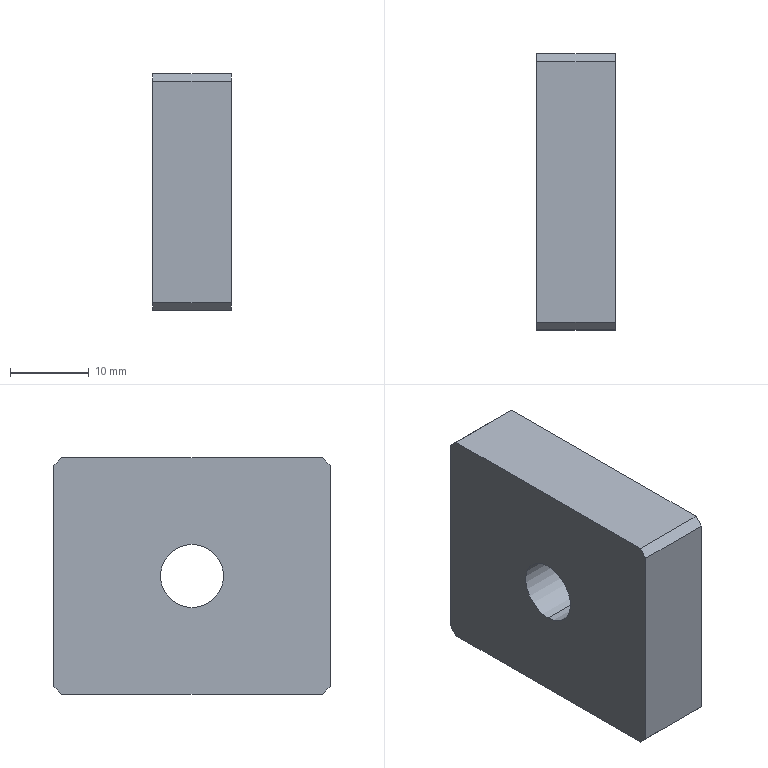Component | SolidWorks | XT-1-19-2-1 | 1 solid | 20 faces | box 10 x 35 x 30 mm | volume 9715 mm3 | plane 10 | cylinder 6 | cone 4 | commonest cylinder face diameters 3.3 x4 8 x2
build123d program:
from build123d import *

# Parameters (mm, degrees)
SKETCH1_W             = 30
SKETCH1_H             = 35
BOSS_EXTRUDE1_DEPTH   = 10
M4_TAPPED_HOLE1_D     = 3.3
M4_TAPPED_HOLE1_DEPTH = 15
M4_TAPPED_HOLE1_TIP   = 0.9914
M8_TAPPED_HOLE1_D     = 8
CHAMFER1_SIZE         = 1


with BuildPart() as part:
    # Sketch1 → Boss-Extrude1 (new body)
    with BuildSketch(Plane.XY):
        with Locations((15, -17.5)):
            Rectangle(SKETCH1_W, SKETCH1_H)
    extrude(amount=BOSS_EXTRUDE1_DEPTH)

    # M4 Tapped Hole1
    with Locations(Plane.ZY):
        with Locations((5, -7.5), (5, -27.5)):
            Hole(M4_TAPPED_HOLE1_D / 2, depth=M4_TAPPED_HOLE1_DEPTH)
            with Locations((0, 0, -(M4_TAPPED_HOLE1_DEPTH + M4_TAPPED_HOLE1_TIP / 2))):  # 118° drill point
                Cone(0, M4_TAPPED_HOLE1_D / 2, M4_TAPPED_HOLE1_TIP, mode=Mode.SUBTRACT)

    # M8 Tapped Hole1 (through all)
    with Locations(Plane.XY.offset(10)):
        with Locations((15, -17.5)):
            Hole(M8_TAPPED_HOLE1_D / 2)

    # Chamfer1
    chamfer1_edges = [part.edges().sort_by_distance(p)[0] for p in [
        (0, 0, 5),
        (30, 0, 5),
        (30, -35, 5),
        (0, -35, 5),
    ]]
    chamfer(chamfer1_edges, length=CHAMFER1_SIZE)


solid = part.part

# Placed as in the assembly
solid = solid.moved(Location((597.283, -101.115, -151), (0, -90, 0)))
STEP:
#1=COLOUR_RGB('',0.7922,0.8196,0.9333);
#2=FILL_AREA_STYLE_COLOUR('',#1);
#3=FILL_AREA_STYLE('',(#2));
#4=SURFACE_STYLE_FILL_AREA(#3);
#5=SURFACE_SIDE_STYLE('',(#4));
#6=SURFACE_STYLE_USAGE(.BOTH.,#5);
#7=PRESENTATION_STYLE_ASSIGNMENT((#6));
#8=CARTESIAN_POINT('',(23.515,-4.67,-5.512));
#9=VERTEX_POINT('',#8);
#10=CARTESIAN_POINT('',(23.515,-4.67,-5.197));
#11=VERTEX_POINT('',#10);
#12=CARTESIAN_POINT('',(23.515,-4.67,-5.354));
#13=DIRECTION('',(-1.,-0.,-0.));
#14=DIRECTION('',(0.,0.,1.));
#15=AXIS2_PLACEMENT_3D('',#12,#13,#14);
#16=CIRCLE('',#15,0.1575);
#17=EDGE_CURVE('',#9,#11,#16,.T.);
#18=ORIENTED_EDGE('',*,*,#17,.F.);
#19=CARTESIAN_POINT('',(23.121,-4.67,-5.512));
#20=VERTEX_POINT('',#19);
#21=CARTESIAN_POINT('',(23.121,-4.67,-5.512));
#22=DIRECTION('',(-1.,-0.,-0.));
#23=VECTOR('',#22,39.37);
#24=LINE('',#21,#23);
#25=EDGE_CURVE('',#9,#20,#24,.T.);
#26=ORIENTED_EDGE('',*,*,#25,.T.);
#27=CARTESIAN_POINT('',(23.121,-4.67,-5.197));
#28=VERTEX_POINT('',#27);
#29=CARTESIAN_POINT('',(23.121,-4.67,-5.354));
#30=DIRECTION('',(-1.,-0.,-0.));
#31=DIRECTION('',(0.,0.,1.));
#32=AXIS2_PLACEMENT_3D('',#29,#30,#31);
#33=CIRCLE('',#32,0.1575);
#34=EDGE_CURVE('',#20,#28,#33,.T.);
#35=ORIENTED_EDGE('',*,*,#34,.T.);
#36=CARTESIAN_POINT('',(23.121,-4.67,-5.197));
#37=DIRECTION('',(-1.,-0.,-0.));
#38=VECTOR('',#37,39.37);
#39=LINE('',#36,#38);
#40=EDGE_CURVE('',#11,#28,#39,.T.);
#41=ORIENTED_EDGE('',*,*,#40,.F.);
#42=EDGE_LOOP('',(#18,#26,#35,#41));
#43=FACE_OUTER_BOUND('',#42,.T.);
#44=CARTESIAN_POINT('',(23.121,-4.67,-5.354));
#45=DIRECTION('',(-1.,-0.,-0.));
#46=DIRECTION('',(0.,0.,1.));
#47=AXIS2_PLACEMENT_3D('',#44,#45,#46);
#48=CYLINDRICAL_SURFACE('',#47,0.1575);
#49=ADVANCED_FACE('',(#43),#48,.F.);
#50=CARTESIAN_POINT('',(23.383,-4.276,-5.354));
#51=VERTEX_POINT('',#50);
#52=CARTESIAN_POINT('',(23.253,-4.276,-5.354));
#53=VERTEX_POINT('',#52);
#54=CARTESIAN_POINT('',(23.318,-4.276,-5.354));
#55=DIRECTION('',(0.,0.,-1.));
#56=DIRECTION('',(-1.,0.,0.));
#57=AXIS2_PLACEMENT_3D('',#54,#55,#56);
#58=CIRCLE('',#57,0.06496);
#59=EDGE_CURVE('',#51,#53,#58,.T.);
#60=ORIENTED_EDGE('',*,*,#59,.F.);
#61=CARTESIAN_POINT('',(23.383,-4.276,-5.945));
#62=VERTEX_POINT('',#61);
#63=CARTESIAN_POINT('',(23.383,-4.276,-5.945));
#64=DIRECTION('',(0.,0.,-1.));
#65=VECTOR('',#64,39.37);
#66=LINE('',#63,#65);
#67=EDGE_CURVE('',#51,#62,#66,.T.);
#68=ORIENTED_EDGE('',*,*,#67,.T.);
#69=CARTESIAN_POINT('',(23.253,-4.276,-5.945));
#70=VERTEX_POINT('',#69);
#71=CARTESIAN_POINT('',(23.318,-4.276,-5.945));
#72=DIRECTION('',(0.,0.,-1.));
#73=DIRECTION('',(-1.,0.,0.));
#74=AXIS2_PLACEMENT_3D('',#71,#72,#73);
#75=CIRCLE('',#74,0.06496);
#76=EDGE_CURVE('',#62,#70,#75,.T.);
#77=ORIENTED_EDGE('',*,*,#76,.T.);
#78=CARTESIAN_POINT('',(23.253,-4.276,-5.945));
#79=DIRECTION('',(0.,0.,-1.));
#80=VECTOR('',#79,39.37);
#81=LINE('',#78,#80);
#82=EDGE_CURVE('',#53,#70,#81,.T.);
#83=ORIENTED_EDGE('',*,*,#82,.F.);
#84=EDGE_LOOP('',(#60,#68,#77,#83));
#85=FACE_OUTER_BOUND('',#84,.T.);
#86=CARTESIAN_POINT('',(23.318,-4.276,-5.945));
#87=DIRECTION('',(0.,0.,-1.));
#88=DIRECTION('',(-1.,0.,0.));
#89=AXIS2_PLACEMENT_3D('',#86,#87,#88);
#90=CYLINDRICAL_SURFACE('',#89,0.06496);
#91=ADVANCED_FACE('',(#85),#90,.F.);
#92=CARTESIAN_POINT('',(23.318,-4.276,-5.315));
#93=VERTEX_POINT('',#92);
#94=CARTESIAN_POINT('',(23.253,-4.276,-5.354));
#95=DIRECTION('',(-0.8572,-0.,-0.515));
#96=VECTOR('',#95,39.37);
#97=LINE('',#94,#96);
#98=EDGE_CURVE('',#93,#53,#97,.T.);
#99=ORIENTED_EDGE('',*,*,#98,.F.);
#100=CARTESIAN_POINT('',(23.383,-4.276,-5.354));
#101=DIRECTION('',(0.8572,0.,-0.515));
#102=VECTOR('',#101,39.37);
#103=LINE('',#100,#102);
#104=EDGE_CURVE('',#93,#51,#103,.T.);
#105=ORIENTED_EDGE('',*,*,#104,.T.);
#106=ORIENTED_EDGE('',*,*,#59,.T.);
#107=EDGE_LOOP('',(#99,#105,#106));
#108=FACE_OUTER_BOUND('',#107,.T.);
#109=CARTESIAN_POINT('',(23.318,-4.276,-5.354));
#110=DIRECTION('',(0.,0.,-1.));
#111=DIRECTION('',(-1.,0.,0.));
#112=AXIS2_PLACEMENT_3D('',#109,#110,#111);
#113=CONICAL_SURFACE('',#112,0.06496,1.03);
#114=ADVANCED_FACE('',(#108),#113,.F.);
#115=CARTESIAN_POINT('',(23.383,-5.064,-5.354));
#116=VERTEX_POINT('',#115);
#117=CARTESIAN_POINT('',(23.253,-5.064,-5.354));
#118=VERTEX_POINT('',#117);
#119=CARTESIAN_POINT('',(23.318,-5.064,-5.354));
#120=DIRECTION('',(0.,0.,-1.));
#121=DIRECTION('',(-1.,0.,0.));
#122=AXIS2_PLACEMENT_3D('',#119,#120,#121);
#123=CIRCLE('',#122,0.06496);
#124=EDGE_CURVE('',#116,#118,#123,.T.);
#125=ORIENTED_EDGE('',*,*,#124,.F.);
#126=CARTESIAN_POINT('',(23.383,-5.064,-5.945));
#127=VERTEX_POINT('',#126);
#128=CARTESIAN_POINT('',(23.383,-5.064,-5.945));
#129=DIRECTION('',(0.,0.,-1.));
#130=VECTOR('',#129,39.37);
#131=LINE('',#128,#130);
#132=EDGE_CURVE('',#116,#127,#131,.T.);
#133=ORIENTED_EDGE('',*,*,#132,.T.);
#134=CARTESIAN_POINT('',(23.253,-5.064,-5.945));
#135=VERTEX_POINT('',#134);
#136=CARTESIAN_POINT('',(23.318,-5.064,-5.945));
#137=DIRECTION('',(0.,0.,-1.));
#138=DIRECTION('',(-1.,0.,0.));
#139=AXIS2_PLACEMENT_3D('',#136,#137,#138);
#140=CIRCLE('',#139,0.06496);
#141=EDGE_CURVE('',#127,#135,#140,.T.);
#142=ORIENTED_EDGE('',*,*,#141,.T.);
#143=CARTESIAN_POINT('',(23.253,-5.064,-5.945));
#144=DIRECTION('',(0.,0.,-1.));
#145=VECTOR('',#144,39.37);
#146=LINE('',#143,#145);
#147=EDGE_CURVE('',#118,#135,#146,.T.);
#148=ORIENTED_EDGE('',*,*,#147,.F.);
#149=EDGE_LOOP('',(#125,#133,#142,#148));
#150=FACE_OUTER_BOUND('',#149,.T.);
#151=CARTESIAN_POINT('',(23.318,-5.064,-5.945));
#152=DIRECTION('',(0.,0.,-1.));
#153=DIRECTION('',(-1.,0.,0.));
#154=AXIS2_PLACEMENT_3D('',#151,#152,#153);
#155=CYLINDRICAL_SURFACE('',#154,0.06496);
#156=ADVANCED_FACE('',(#150),#155,.F.);
#157=CARTESIAN_POINT('',(23.318,-5.064,-5.315));
#158=VERTEX_POINT('',#157);
#159=CARTESIAN_POINT('',(23.253,-5.064,-5.354));
#160=DIRECTION('',(-0.8572,-0.,-0.515));
#161=VECTOR('',#160,39.37);
#162=LINE('',#159,#161);
#163=EDGE_CURVE('',#158,#118,#162,.T.);
#164=ORIENTED_EDGE('',*,*,#163,.F.);
#165=CARTESIAN_POINT('',(23.383,-5.064,-5.354));
#166=DIRECTION('',(0.8572,0.,-0.515));
#167=VECTOR('',#166,39.37);
#168=LINE('',#165,#167);
#169=EDGE_CURVE('',#158,#116,#168,.T.);
#170=ORIENTED_EDGE('',*,*,#169,.T.);
#171=ORIENTED_EDGE('',*,*,#124,.T.);
#172=EDGE_LOOP('',(#164,#170,#171));
#173=FACE_OUTER_BOUND('',#172,.T.);
#174=CARTESIAN_POINT('',(23.318,-5.064,-5.354));
#175=DIRECTION('',(0.,0.,-1.));
#176=DIRECTION('',(-1.,0.,0.));
#177=AXIS2_PLACEMENT_3D('',#174,#175,#176);
#178=CONICAL_SURFACE('',#177,0.06496,1.03);
#179=ADVANCED_FACE('',(#173),#178,.F.);
#180=CARTESIAN_POINT('',(23.318,-4.276,-5.945));
#181=DIRECTION('',(0.,0.,-1.));
#182=DIRECTION('',(-1.,0.,0.));
#183=AXIS2_PLACEMENT_3D('',#180,#181,#182);
#184=CIRCLE('',#183,0.06496);
#185=EDGE_CURVE('',#70,#62,#184,.T.);
#186=ORIENTED_EDGE('',*,*,#185,.F.);
#187=ORIENTED_EDGE('',*,*,#76,.F.);
#188=EDGE_LOOP('',(#186,#187));
#189=FACE_BOUND('',#188,.T.);
#190=CARTESIAN_POINT('',(23.318,-5.064,-5.945));
#191=DIRECTION('',(0.,0.,-1.));
#192=DIRECTION('',(-1.,0.,0.));
#193=AXIS2_PLACEMENT_3D('',#190,#191,#192);
#194=CIRCLE('',#193,0.06496);
#195=EDGE_CURVE('',#135,#127,#194,.T.);
#196=ORIENTED_EDGE('',*,*,#195,.F.);
#197=ORIENTED_EDGE('',*,*,#141,.F.);
#198=EDGE_LOOP('',(#196,#197));
#199=FACE_BOUND('',#198,.T.);
#200=CARTESIAN_POINT('',(23.121,-4.02,-5.945));
#201=VERTEX_POINT('',#200);
#202=CARTESIAN_POINT('',(23.121,-5.319,-5.945));
#203=VERTEX_POINT('',#202);
#204=CARTESIAN_POINT('',(23.121,-3.981,-5.945));
#205=DIRECTION('',(0.,-1.,0.));
#206=VECTOR('',#205,39.37);
#207=LINE('',#204,#206);
#208=EDGE_CURVE('',#201,#203,#207,.T.);
#209=ORIENTED_EDGE('',*,*,#208,.F.);
#210=CARTESIAN_POINT('',(23.515,-4.02,-5.945));
#211=VERTEX_POINT('',#210);
#212=CARTESIAN_POINT('',(23.121,-4.02,-5.945));
#213=DIRECTION('',(1.,0.,0.));
#214=VECTOR('',#213,39.37);
#215=LINE('',#212,#214);
#216=EDGE_CURVE('',#201,#211,#215,.T.);
#217=ORIENTED_EDGE('',*,*,#216,.T.);
#218=CARTESIAN_POINT('',(23.515,-5.319,-5.945));
#219=VERTEX_POINT('',#218);
#220=CARTESIAN_POINT('',(23.515,-3.981,-5.945));
#221=DIRECTION('',(0.,-1.,0.));
#222=VECTOR('',#221,39.37);
#223=LINE('',#220,#222);
#224=EDGE_CURVE('',#211,#219,#223,.T.);
#225=ORIENTED_EDGE('',*,*,#224,.T.);
#226=CARTESIAN_POINT('',(23.121,-5.319,-5.945));
#227=DIRECTION('',(-1.,-0.,-0.));
#228=VECTOR('',#227,39.37);
#229=LINE('',#226,#228);
#230=EDGE_CURVE('',#219,#203,#229,.T.);
#231=ORIENTED_EDGE('',*,*,#230,.T.);
#232=EDGE_LOOP('',(#209,#217,#225,#231));
#233=FACE_OUTER_BOUND('',#232,.T.);
#234=CARTESIAN_POINT('',(23.121,-3.981,-5.945));
#235=DIRECTION('',(-0.,0.,1.));
#236=DIRECTION('',(-0.,1.,-0.));
#237=AXIS2_PLACEMENT_3D('',#234,#235,#236);
#238=PLANE('',#237);
#239=ADVANCED_FACE('',(#189,#199,#233),#238,.F.);
#240=CARTESIAN_POINT('',(23.515,-5.359,-5.906));
#241=VERTEX_POINT('',#240);
#242=CARTESIAN_POINT('',(23.515,-5.359,-4.803));
#243=VERTEX_POINT('',#242);
#244=CARTESIAN_POINT('',(23.515,-5.359,-5.945));
#245=DIRECTION('',(-0.,-0.,1.));
#246=VECTOR('',#245,39.37);
#247=LINE('',#244,#246);
#248=EDGE_CURVE('',#241,#243,#247,.T.);
#249=ORIENTED_EDGE('',*,*,#248,.T.);
#250=CARTESIAN_POINT('',(23.121,-5.359,-4.803));
#251=VERTEX_POINT('',#250);
#252=CARTESIAN_POINT('',(23.121,-5.359,-4.803));
#253=DIRECTION('',(-1.,-0.,-0.));
#254=VECTOR('',#253,39.37);
#255=LINE('',#252,#254);
#256=EDGE_CURVE('',#243,#251,#255,.T.);
#257=ORIENTED_EDGE('',*,*,#256,.T.);
#258=CARTESIAN_POINT('',(23.121,-5.359,-5.906));
#259=VERTEX_POINT('',#258);
#260=CARTESIAN_POINT('',(23.121,-5.359,-5.945));
#261=DIRECTION('',(-0.,-0.,1.));
#262=VECTOR('',#261,39.37);
#263=LINE('',#260,#262);
#264=EDGE_CURVE('',#259,#251,#263,.T.);
#265=ORIENTED_EDGE('',*,*,#264,.F.);
#266=CARTESIAN_POINT('',(23.121,-5.359,-5.906));
#267=DIRECTION('',(1.,0.,0.));
#268=VECTOR('',#267,39.37);
#269=LINE('',#266,#268);
#270=EDGE_CURVE('',#259,#241,#269,.T.);
#271=ORIENTED_EDGE('',*,*,#270,.T.);
#272=EDGE_LOOP('',(#249,#257,#265,#271));
#273=FACE_OUTER_BOUND('',#272,.T.);
#274=CARTESIAN_POINT('',(23.121,-5.359,-5.945));
#275=DIRECTION('',(-0.,1.,0.));
#276=DIRECTION('',(-1.,-0.,-0.));
#277=AXIS2_PLACEMENT_3D('',#274,#275,#276);
#278=PLANE('',#277);
#279=ADVANCED_FACE('',(#273),#278,.F.);
#280=CARTESIAN_POINT('',(23.515,-5.319,-4.764));
#281=VERTEX_POINT('',#280);
#282=CARTESIAN_POINT('',(23.515,-4.02,-4.764));
#283=VERTEX_POINT('',#282);
#284=CARTESIAN_POINT('',(23.515,-3.981,-4.764));
#285=DIRECTION('',(-0.,1.,0.));
#286=VECTOR('',#285,39.37);
#287=LINE('',#284,#286);
#288=EDGE_CURVE('',#281,#283,#287,.T.);
#289=ORIENTED_EDGE('',*,*,#288,.T.);
#290=CARTESIAN_POINT('',(23.121,-4.02,-4.764));
#291=VERTEX_POINT('',#290);
#292=CARTESIAN_POINT('',(23.121,-4.02,-4.764));
#293=DIRECTION('',(-1.,-0.,-0.));
#294=VECTOR('',#293,39.37);
#295=LINE('',#292,#294);
#296=EDGE_CURVE('',#283,#291,#295,.T.);
#297=ORIENTED_EDGE('',*,*,#296,.T.);
#298=CARTESIAN_POINT('',(23.121,-5.319,-4.764));
#299=VERTEX_POINT('',#298);
#300=CARTESIAN_POINT('',(23.121,-3.981,-4.764));
#301=DIRECTION('',(-0.,1.,0.));
#302=VECTOR('',#301,39.37);
#303=LINE('',#300,#302);
#304=EDGE_CURVE('',#299,#291,#303,.T.);
#305=ORIENTED_EDGE('',*,*,#304,.F.);
#306=CARTESIAN_POINT('',(23.121,-5.319,-4.764));
#307=DIRECTION('',(1.,0.,0.));
#308=VECTOR('',#307,39.37);
#309=LINE('',#306,#308);
#310=EDGE_CURVE('',#299,#281,#309,.T.);
#311=ORIENTED_EDGE('',*,*,#310,.T.);
#312=EDGE_LOOP('',(#289,#297,#305,#311));
#313=FACE_OUTER_BOUND('',#312,.T.);
#314=CARTESIAN_POINT('',(23.121,-3.981,-4.764));
#315=DIRECTION('',(0.,0.,-1.));
#316=DIRECTION('',(0.,-1.,-0.));
#317=AXIS2_PLACEMENT_3D('',#314,#315,#316);
#318=PLANE('',#317);
#319=ADVANCED_FACE('',(#313),#318,.F.);
#320=CARTESIAN_POINT('',(23.515,-3.981,-4.803));
#321=VERTEX_POINT('',#320);
#322=CARTESIAN_POINT('',(23.515,-3.981,-5.906));
#323=VERTEX_POINT('',#322);
#324=CARTESIAN_POINT('',(23.515,-3.981,-5.945));
#325=DIRECTION('',(0.,0.,-1.));
#326=VECTOR('',#325,39.37);
#327=LINE('',#324,#326);
#328=EDGE_CURVE('',#321,#323,#327,.T.);
#329=ORIENTED_EDGE('',*,*,#328,.T.);
#330=CARTESIAN_POINT('',(23.121,-3.981,-5.906));
#331=VERTEX_POINT('',#330);
#332=CARTESIAN_POINT('',(23.121,-3.981,-5.906));
#333=DIRECTION('',(-1.,-0.,-0.));
#334=VECTOR('',#333,39.37);
#335=LINE('',#332,#334);
#336=EDGE_CURVE('',#323,#331,#335,.T.);
#337=ORIENTED_EDGE('',*,*,#336,.T.);
#338=CARTESIAN_POINT('',(23.121,-3.981,-4.803));
#339=VERTEX_POINT('',#338);
#340=CARTESIAN_POINT('',(23.121,-3.981,-5.945));
#341=DIRECTION('',(0.,0.,-1.));
#342=VECTOR('',#341,39.37);
#343=LINE('',#340,#342);
#344=EDGE_CURVE('',#339,#331,#343,.T.);
#345=ORIENTED_EDGE('',*,*,#344,.F.);
#346=CARTESIAN_POINT('',(23.121,-3.981,-4.803));
#347=DIRECTION('',(1.,0.,0.));
#348=VECTOR('',#347,39.37);
#349=LINE('',#346,#348);
#350=EDGE_CURVE('',#339,#321,#349,.T.);
#351=ORIENTED_EDGE('',*,*,#350,.T.);
#352=EDGE_LOOP('',(#329,#337,#345,#351));
#353=FACE_OUTER_BOUND('',#352,.T.);
#354=CARTESIAN_POINT('',(23.121,-3.981,-5.945));
#355=DIRECTION('',(0.,-1.,-0.));
#356=DIRECTION('',(1.,0.,0.));
#357=AXIS2_PLACEMENT_3D('',#354,#355,#356);
#358=PLANE('',#357);
#359=ADVANCED_FACE('',(#353),#358,.F.);
#360=CARTESIAN_POINT('',(23.121,-4.67,-5.354));
#361=DIRECTION('',(-1.,-0.,-0.));
#362=DIRECTION('',(0.,0.,1.));
#363=AXIS2_PLACEMENT_3D('',#360,#361,#362);
#364=CIRCLE('',#363,0.1575);
#365=EDGE_CURVE('',#28,#20,#364,.T.);
#366=ORIENTED_EDGE('',*,*,#365,.F.);
#367=ORIENTED_EDGE('',*,*,#34,.F.);
#368=EDGE_LOOP('',(#366,#367));
#369=FACE_BOUND('',#368,.T.);
#370=ORIENTED_EDGE('',*,*,#344,.T.);
#371=CARTESIAN_POINT('',(23.121,-4.001,-5.925));
#372=DIRECTION('',(0.,-0.7071,-0.7071));
#373=VECTOR('',#372,39.37);
#374=LINE('',#371,#373);
#375=EDGE_CURVE('',#331,#201,#374,.T.);
#376=ORIENTED_EDGE('',*,*,#375,.T.);
#377=ORIENTED_EDGE('',*,*,#208,.T.);
#378=CARTESIAN_POINT('',(23.121,-4.65,-6.614));
#379=DIRECTION('',(0.,-0.7071,0.7071));
#380=VECTOR('',#379,39.37);
#381=LINE('',#378,#380);
#382=EDGE_CURVE('',#203,#259,#381,.T.);
#383=ORIENTED_EDGE('',*,*,#382,.T.);
#384=ORIENTED_EDGE('',*,*,#264,.T.);
#385=CARTESIAN_POINT('',(23.121,-5.241,-4.685));
#386=DIRECTION('',(-0.,0.7071,0.7071));
#387=VECTOR('',#386,39.37);
#388=LINE('',#385,#387);
#389=EDGE_CURVE('',#251,#299,#388,.T.);
#390=ORIENTED_EDGE('',*,*,#389,.T.);
#391=ORIENTED_EDGE('',*,*,#304,.T.);
#392=CARTESIAN_POINT('',(23.121,-3.41,-5.374));
#393=DIRECTION('',(-0.,0.7071,-0.7071));
#394=VECTOR('',#393,39.37);
#395=LINE('',#392,#394);
#396=EDGE_CURVE('',#291,#339,#395,.T.);
#397=ORIENTED_EDGE('',*,*,#396,.T.);
#398=EDGE_LOOP('',(#370,#376,#377,#383,#384,#390,#391,#397));
#399=FACE_OUTER_BOUND('',#398,.T.);
#400=CARTESIAN_POINT('',(23.121,-3.981,-5.945));
#401=DIRECTION('',(-1.,-0.,-0.));
#402=DIRECTION('',(-0.,-0.,1.));
#403=AXIS2_PLACEMENT_3D('',#400,#401,#402);
#404=PLANE('',#403);
#405=ADVANCED_FACE('',(#369,#399),#404,.T.);
#406=CARTESIAN_POINT('',(23.515,-4.67,-5.354));
#407=DIRECTION('',(-1.,-0.,-0.));
#408=DIRECTION('',(0.,0.,1.));
#409=AXIS2_PLACEMENT_3D('',#406,#407,#408);
#410=CIRCLE('',#409,0.1575);
#411=EDGE_CURVE('',#11,#9,#410,.T.);
#412=ORIENTED_EDGE('',*,*,#411,.T.);
#413=ORIENTED_EDGE('',*,*,#17,.T.);
#414=EDGE_LOOP('',(#412,#413));
#415=FACE_BOUND('',#414,.T.);
#416=ORIENTED_EDGE('',*,*,#224,.F.);
#417=CARTESIAN_POINT('',(23.515,-4.02,-5.945));
#418=DIRECTION('',(-0.,0.7071,0.7071));
#419=VECTOR('',#418,39.37);
#420=LINE('',#417,#419);
#421=EDGE_CURVE('',#211,#323,#420,.T.);
#422=ORIENTED_EDGE('',*,*,#421,.T.);
#423=ORIENTED_EDGE('',*,*,#328,.F.);
#424=CARTESIAN_POINT('',(23.515,-3.981,-4.803));
#425=DIRECTION('',(0.,-0.7071,0.7071));
#426=VECTOR('',#425,39.37);
#427=LINE('',#424,#426);
#428=EDGE_CURVE('',#321,#283,#427,.T.);
#429=ORIENTED_EDGE('',*,*,#428,.T.);
#430=ORIENTED_EDGE('',*,*,#288,.F.);
#431=CARTESIAN_POINT('',(23.515,-5.319,-4.764));
#432=DIRECTION('',(0.,-0.7071,-0.7071));
#433=VECTOR('',#432,39.37);
#434=LINE('',#431,#433);
#435=EDGE_CURVE('',#281,#243,#434,.T.);
#436=ORIENTED_EDGE('',*,*,#435,.T.);
#437=ORIENTED_EDGE('',*,*,#248,.F.);
#438=CARTESIAN_POINT('',(23.515,-5.359,-5.906));
#439=DIRECTION('',(-0.,0.7071,-0.7071));
#440=VECTOR('',#439,39.37);
#441=LINE('',#438,#440);
#442=EDGE_CURVE('',#241,#219,#441,.T.);
#443=ORIENTED_EDGE('',*,*,#442,.T.);
#444=EDGE_LOOP('',(#416,#422,#423,#429,#430,#436,#437,#443));
#445=FACE_OUTER_BOUND('',#444,.T.);
#446=CARTESIAN_POINT('',(23.515,-3.981,-5.945));
#447=DIRECTION('',(-1.,-0.,-0.));
#448=DIRECTION('',(-0.,-0.,1.));
#449=AXIS2_PLACEMENT_3D('',#446,#447,#448);
#450=PLANE('',#449);
#451=ADVANCED_FACE('',(#415,#445),#450,.F.);
#452=ORIENTED_EDGE('',*,*,#169,.F.);
#453=ORIENTED_EDGE('',*,*,#163,.T.);
#454=CARTESIAN_POINT('',(23.318,-5.064,-5.354));
#455=DIRECTION('',(0.,0.,-1.));
#456=DIRECTION('',(-1.,0.,0.));
#457=AXIS2_PLACEMENT_3D('',#454,#455,#456);
#458=CIRCLE('',#457,0.06496);
#459=EDGE_CURVE('',#118,#116,#458,.T.);
#460=ORIENTED_EDGE('',*,*,#459,.T.);
#461=EDGE_LOOP('',(#452,#453,#460));
#462=FACE_OUTER_BOUND('',#461,.T.);
#463=CARTESIAN_POINT('',(23.318,-5.064,-5.354));
#464=DIRECTION('',(0.,0.,-1.));
#465=DIRECTION('',(-1.,0.,0.));
#466=AXIS2_PLACEMENT_3D('',#463,#464,#465);
#467=CONICAL_SURFACE('',#466,0.06496,1.03);
#468=ADVANCED_FACE('',(#462),#467,.F.);
#469=ORIENTED_EDGE('',*,*,#132,.F.);
#470=ORIENTED_EDGE('',*,*,#459,.F.);
#471=ORIENTED_EDGE('',*,*,#147,.T.);
#472=ORIENTED_EDGE('',*,*,#195,.T.);
#473=EDGE_LOOP('',(#469,#470,#471,#472));
#474=FACE_OUTER_BOUND('',#473,.T.);
#475=CARTESIAN_POINT('',(23.318,-5.064,-5.945));
#476=DIRECTION('',(0.,0.,-1.));
#477=DIRECTION('',(-1.,0.,0.));
#478=AXIS2_PLACEMENT_3D('',#475,#476,#477);
#479=CYLINDRICAL_SURFACE('',#478,0.06496);
#480=ADVANCED_FACE('',(#474),#479,.F.);
#481=ORIENTED_EDGE('',*,*,#104,.F.);
#482=ORIENTED_EDGE('',*,*,#98,.T.);
#483=CARTESIAN_POINT('',(23.318,-4.276,-5.354));
#484=DIRECTION('',(0.,0.,-1.));
#485=DIRECTION('',(-1.,0.,0.));
#486=AXIS2_PLACEMENT_3D('',#483,#484,#485);
#487=CIRCLE('',#486,0.06496);
#488=EDGE_CURVE('',#53,#51,#487,.T.);
#489=ORIENTED_EDGE('',*,*,#488,.T.);
#490=EDGE_LOOP('',(#481,#482,#489));
#491=FACE_OUTER_BOUND('',#490,.T.);
#492=CARTESIAN_POINT('',(23.318,-4.276,-5.354));
#493=DIRECTION('',(0.,0.,-1.));
#494=DIRECTION('',(-1.,0.,0.));
#495=AXIS2_PLACEMENT_3D('',#492,#493,#494);
#496=CONICAL_SURFACE('',#495,0.06496,1.03);
#497=ADVANCED_FACE('',(#491),#496,.F.);
#498=ORIENTED_EDGE('',*,*,#67,.F.);
#499=ORIENTED_EDGE('',*,*,#488,.F.);
#500=ORIENTED_EDGE('',*,*,#82,.T.);
#501=ORIENTED_EDGE('',*,*,#185,.T.);
#502=EDGE_LOOP('',(#498,#499,#500,#501));
#503=FACE_OUTER_BOUND('',#502,.T.);
#504=CARTESIAN_POINT('',(23.318,-4.276,-5.945));
#505=DIRECTION('',(0.,0.,-1.));
#506=DIRECTION('',(-1.,0.,0.));
#507=AXIS2_PLACEMENT_3D('',#504,#505,#506);
#508=CYLINDRICAL_SURFACE('',#507,0.06496);
#509=ADVANCED_FACE('',(#503),#508,.F.);
#510=ORIENTED_EDGE('',*,*,#25,.F.);
#511=ORIENTED_EDGE('',*,*,#411,.F.);
#512=ORIENTED_EDGE('',*,*,#40,.T.);
#513=ORIENTED_EDGE('',*,*,#365,.T.);
#514=EDGE_LOOP('',(#510,#511,#512,#513));
#515=FACE_OUTER_BOUND('',#514,.T.);
#516=CARTESIAN_POINT('',(23.121,-4.67,-5.354));
#517=DIRECTION('',(-1.,-0.,-0.));
#518=DIRECTION('',(0.,0.,1.));
#519=AXIS2_PLACEMENT_3D('',#516,#517,#518);
#520=CYLINDRICAL_SURFACE('',#519,0.1575);
#521=ADVANCED_FACE('',(#515),#520,.F.);
#522=ORIENTED_EDGE('',*,*,#375,.F.);
#523=ORIENTED_EDGE('',*,*,#336,.F.);
#524=ORIENTED_EDGE('',*,*,#421,.F.);
#525=ORIENTED_EDGE('',*,*,#216,.F.);
#526=EDGE_LOOP('',(#522,#523,#524,#525));
#527=FACE_OUTER_BOUND('',#526,.T.);
#528=CARTESIAN_POINT('',(23.121,-4.02,-5.945));
#529=DIRECTION('',(0.,-0.7071,0.7071));
#530=DIRECTION('',(1.,0.,0.));
#531=AXIS2_PLACEMENT_3D('',#528,#529,#530);
#532=PLANE('',#531);
#533=ADVANCED_FACE('',(#527),#532,.F.);
#534=ORIENTED_EDGE('',*,*,#396,.F.);
#535=ORIENTED_EDGE('',*,*,#296,.F.);
#536=ORIENTED_EDGE('',*,*,#428,.F.);
#537=ORIENTED_EDGE('',*,*,#350,.F.);
#538=EDGE_LOOP('',(#534,#535,#536,#537));
#539=FACE_OUTER_BOUND('',#538,.T.);
#540=CARTESIAN_POINT('',(23.121,-3.981,-4.803));
#541=DIRECTION('',(0.,-0.7071,-0.7071));
#542=DIRECTION('',(1.,0.,0.));
#543=AXIS2_PLACEMENT_3D('',#540,#541,#542);
#544=PLANE('',#543);
#545=ADVANCED_FACE('',(#539),#544,.F.);
#546=ORIENTED_EDGE('',*,*,#389,.F.);
#547=ORIENTED_EDGE('',*,*,#256,.F.);
#548=ORIENTED_EDGE('',*,*,#435,.F.);
#549=ORIENTED_EDGE('',*,*,#310,.F.);
#550=EDGE_LOOP('',(#546,#547,#548,#549));
#551=FACE_OUTER_BOUND('',#550,.T.);
#552=CARTESIAN_POINT('',(23.121,-5.319,-4.764));
#553=DIRECTION('',(-0.,0.7071,-0.7071));
#554=DIRECTION('',(1.,0.,0.));
#555=AXIS2_PLACEMENT_3D('',#552,#553,#554);
#556=PLANE('',#555);
#557=ADVANCED_FACE('',(#551),#556,.F.);
#558=ORIENTED_EDGE('',*,*,#382,.F.);
#559=ORIENTED_EDGE('',*,*,#230,.F.);
#560=ORIENTED_EDGE('',*,*,#442,.F.);
#561=ORIENTED_EDGE('',*,*,#270,.F.);
#562=EDGE_LOOP('',(#558,#559,#560,#561));
#563=FACE_OUTER_BOUND('',#562,.T.);
#564=CARTESIAN_POINT('',(23.121,-5.359,-5.906));
#565=DIRECTION('',(-0.,0.7071,0.7071));
#566=DIRECTION('',(1.,0.,0.));
#567=AXIS2_PLACEMENT_3D('',#564,#565,#566);
#568=PLANE('',#567);
#569=ADVANCED_FACE('',(#563),#568,.F.);
#570=CLOSED_SHELL('',(#49,#91,#114,#156,#179,#239,#279,#319,#359,#405,#451,#468,#480,#497,#509,#521,#533,#545,#557,#569));
#571=MANIFOLD_SOLID_BREP('',#570);
#572=STYLED_ITEM('',(#7),#571);
#573=(LENGTH_UNIT()NAMED_UNIT(*)SI_UNIT($,.METRE.));
#574=LENGTH_MEASURE_WITH_UNIT(LENGTH_MEASURE(0.0254),#573);
#575=DIMENSIONAL_EXPONENTS(1.,0.,0.,0.,0.,0.,0.);
#576=(CONVERSION_BASED_UNIT('',#574)LENGTH_UNIT()NAMED_UNIT(#575));
#577=UNCERTAINTY_MEASURE_WITH_UNIT(LENGTH_MEASURE(0.00001),#576,'','');
#578=(NAMED_UNIT(*)PLANE_ANGLE_UNIT()SI_UNIT($,.RADIAN.));
#579=(NAMED_UNIT(*)SI_UNIT($,.STERADIAN.)SOLID_ANGLE_UNIT());
#580=(GEOMETRIC_REPRESENTATION_CONTEXT(3)GLOBAL_UNCERTAINTY_ASSIGNED_CONTEXT((#577))GLOBAL_UNIT_ASSIGNED_CONTEXT((#576,#578,#579))REPRESENTATION_CONTEXT('',''));
#581=MECHANICAL_DESIGN_GEOMETRIC_PRESENTATION_REPRESENTATION('',(#572),#580);
#582=PRESENTATION_LAYER_ASSIGNMENT('','',(#572));
#583=CARTESIAN_POINT('',(0.,0.,0.));
#584=DIRECTION('',(0.,0.,1.));
#585=DIRECTION('',(1.,0.,0.));
#586=AXIS2_PLACEMENT_3D('',#583,#584,#585);
#587=(LENGTH_UNIT()NAMED_UNIT(*)SI_UNIT($,.METRE.));
#588=LENGTH_MEASURE_WITH_UNIT(LENGTH_MEASURE(0.0254),#587);
#589=DIMENSIONAL_EXPONENTS(1.,0.,0.,0.,0.,0.,0.);
#590=(CONVERSION_BASED_UNIT('',#588)LENGTH_UNIT()NAMED_UNIT(#589));
#591=UNCERTAINTY_MEASURE_WITH_UNIT(LENGTH_MEASURE(0.00001),#590,'','');
#592=(NAMED_UNIT(*)PLANE_ANGLE_UNIT()SI_UNIT($,.RADIAN.));
#593=(NAMED_UNIT(*)SI_UNIT($,.STERADIAN.)SOLID_ANGLE_UNIT());
#594=(GEOMETRIC_REPRESENTATION_CONTEXT(3)GLOBAL_UNCERTAINTY_ASSIGNED_CONTEXT((#591))GLOBAL_UNIT_ASSIGNED_CONTEXT((#590,#592,#593))REPRESENTATION_CONTEXT('',''));
#595=ADVANCED_BREP_SHAPE_REPRESENTATION('',(#571,#586),#594);